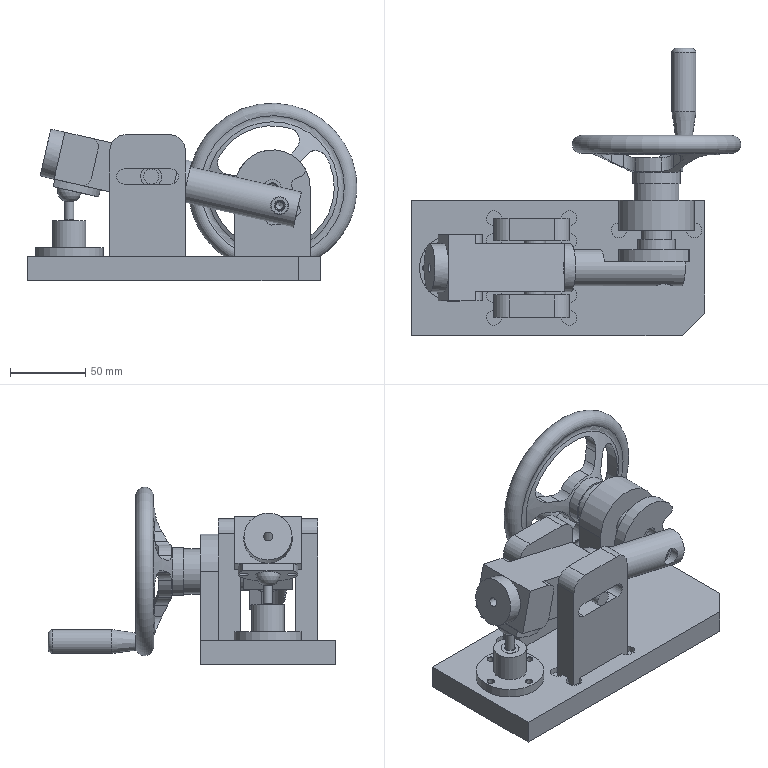Assembly | NX | mm | 14 component files | 14 solids | 336 faces | box 219 x 191 x 118 mm | volume 671878 mm3 | cylinder 145 | plane 140 | cone 40 | torus 5 | sphere 4 | spline 2 | commonest cylinder face diameters 12 x28 10 x20 16 x15 6.5 x8 14 x8 11 x7 6.8 x7 8.5 x7
Bill of materials:
unnamed part 1 | 1 |  | Cylindrical pin with a half-diameter flat cut (D/half-round section) along roughly half its length at one end, and a transverse round hole through the cut end.
unnamed part 2 | 1 |  | Handwheel: round rim with a rounded cross-section, joined to an offset central hub by three spokes, with a central bore and one small hole in the rim.
unnamed part 3 | 1 |  | Stepped cylindrical shaft/spigot with four diameter sections, including a wider collar, a small axial hole in the smaller end, and a center hole with a conical bottom in the opposite end face.
unnamed part 4 | 1 |  | Flanged bushing: a circular flange with four equally spaced through holes, and a cylindrical boss with a central through bore.
unnamed part 5 | 1 |  | Tapered grip/handle with a rounded closed end, a conical transition, a short reduced neck, and an externally grooved (thread-like) stud at the narrow end.
unnamed part 6 | 2 |  | Flat rectangular plate of uniform thickness with two rounded corners at one end and one straight oblong slot through the plate near that end.
unnamed part 7 | 1 |  | Block-shaped body with coaxial cylindrical ends: one end is a hollow cylindrical spigot, the other a cylindrical boss with a small hole. Two collared cylindrical pins stick out from opposite sides.
unnamed part 8 | 1 |  | Flat profiled plate with a large arc-shaped edge, a narrower tab-like lower portion, a through hole, and a second hole, with cylindrical bosses on both faces.
unnamed part 9 | 1 |  | Flanged sleeve bushing: a cylindrical body with a larger-diameter flange at one end, a central through bore, and chamfered outer edges.
unnamed part 10 | 1 |  | D-shaped flange plate (circular with one straight edge) with a central domed boss containing a through bore, and two through holes on either side of the boss.
unnamed part 11 | 1 |  | Rectangular plate with one chamfered corner and a pattern of through holes, including a central hole with four surrounding holes. The top face has shallow recesses: a circular-arc pocket, slot-shaped pockets connecting holes, and a stepped edge region.
unnamed part 12 | 1 |  | Ball stud: a sphere on a slender cylindrical neck, joined at a shoulder to a larger cylindrical shank.
unnamed part 13 | 1 |  | Thick flat plate with a rectangular lower section and a semicircular rounded top end (tab/lug-like profile), with a single circular through-hole near the rounded end.
Mates:
1. center | base_plate 1 face | base_plate 1 face | assembly datumplane
2. center | base_plate 1 face | base_plate 1 face | assembly datumplane
3. touch align | assembly datumplane | base_plate 1 face
4. concentric | base_plate 1 edge | bracket_2 2 edge
5. touch align | bracket_2 2 face | base_plate 1 face
6. touch align | bracket_2 1 face | base_plate 1 face
7. concentric | bracket_2 1 edge | base_plate 1 edge
8. concentric | guide_sleeve 1 edge | base_plate 1 edge
9. touch align | bracket_1 1 face | base_plate 1 face
10. touch align | guide_post 1 face | guide_sleeve 1 face
11. touch align | guide_sleeve 1 face | guide_post 1 face
12. touch align | swing_rod 1 face | swing_part 1 face
13. center | bracket_2 2 face | bracket_2 1 face | swing_part 1 face | swing_part 1 face
14. touch align | crank 1 face | swing_rod 1 face
15. touch align | crank 1 face | bracket_1 1 face
16. touch align | rot_shaft 1 face | bracket_1 1 face
17. touch align | handwheel 1 face | rot_shaft 1 face
18. touch align | handwheel 1 face | rot_shaft 1 face
19. touch align | rot_shaft 1 face | handwheel 1 edge
20. touch align | rot_shaft 1 face | crank 1 face
21. touch align | rot_shaft 1 face | crank 1 edge
22. touch align | crank 1 face | rot_shaft 1 face
23. touch align | crank 1 face | swing_rod 1 face
24. touch align | handle 1 face | handwheel 1 face
25. touch align | handle 1 face | handwheel 1 face
26. touch align | baffle 1 face | swing_rod 1 face
27. touch align | baffle 1 face | swing_rod 1 face
28. touch align | bracket_1 1 face | base_plate 1 face
29. touch align | bracket_1 1 face | base_plate 1 face
30. touch align | cover 1 face | swing_part 1 face
31. touch align | cover 1 face | swing_part 1 face
32. touch align | cover 1 face | swing_part 1 face
33. touch align | cover 1 face | guide_post 1 face